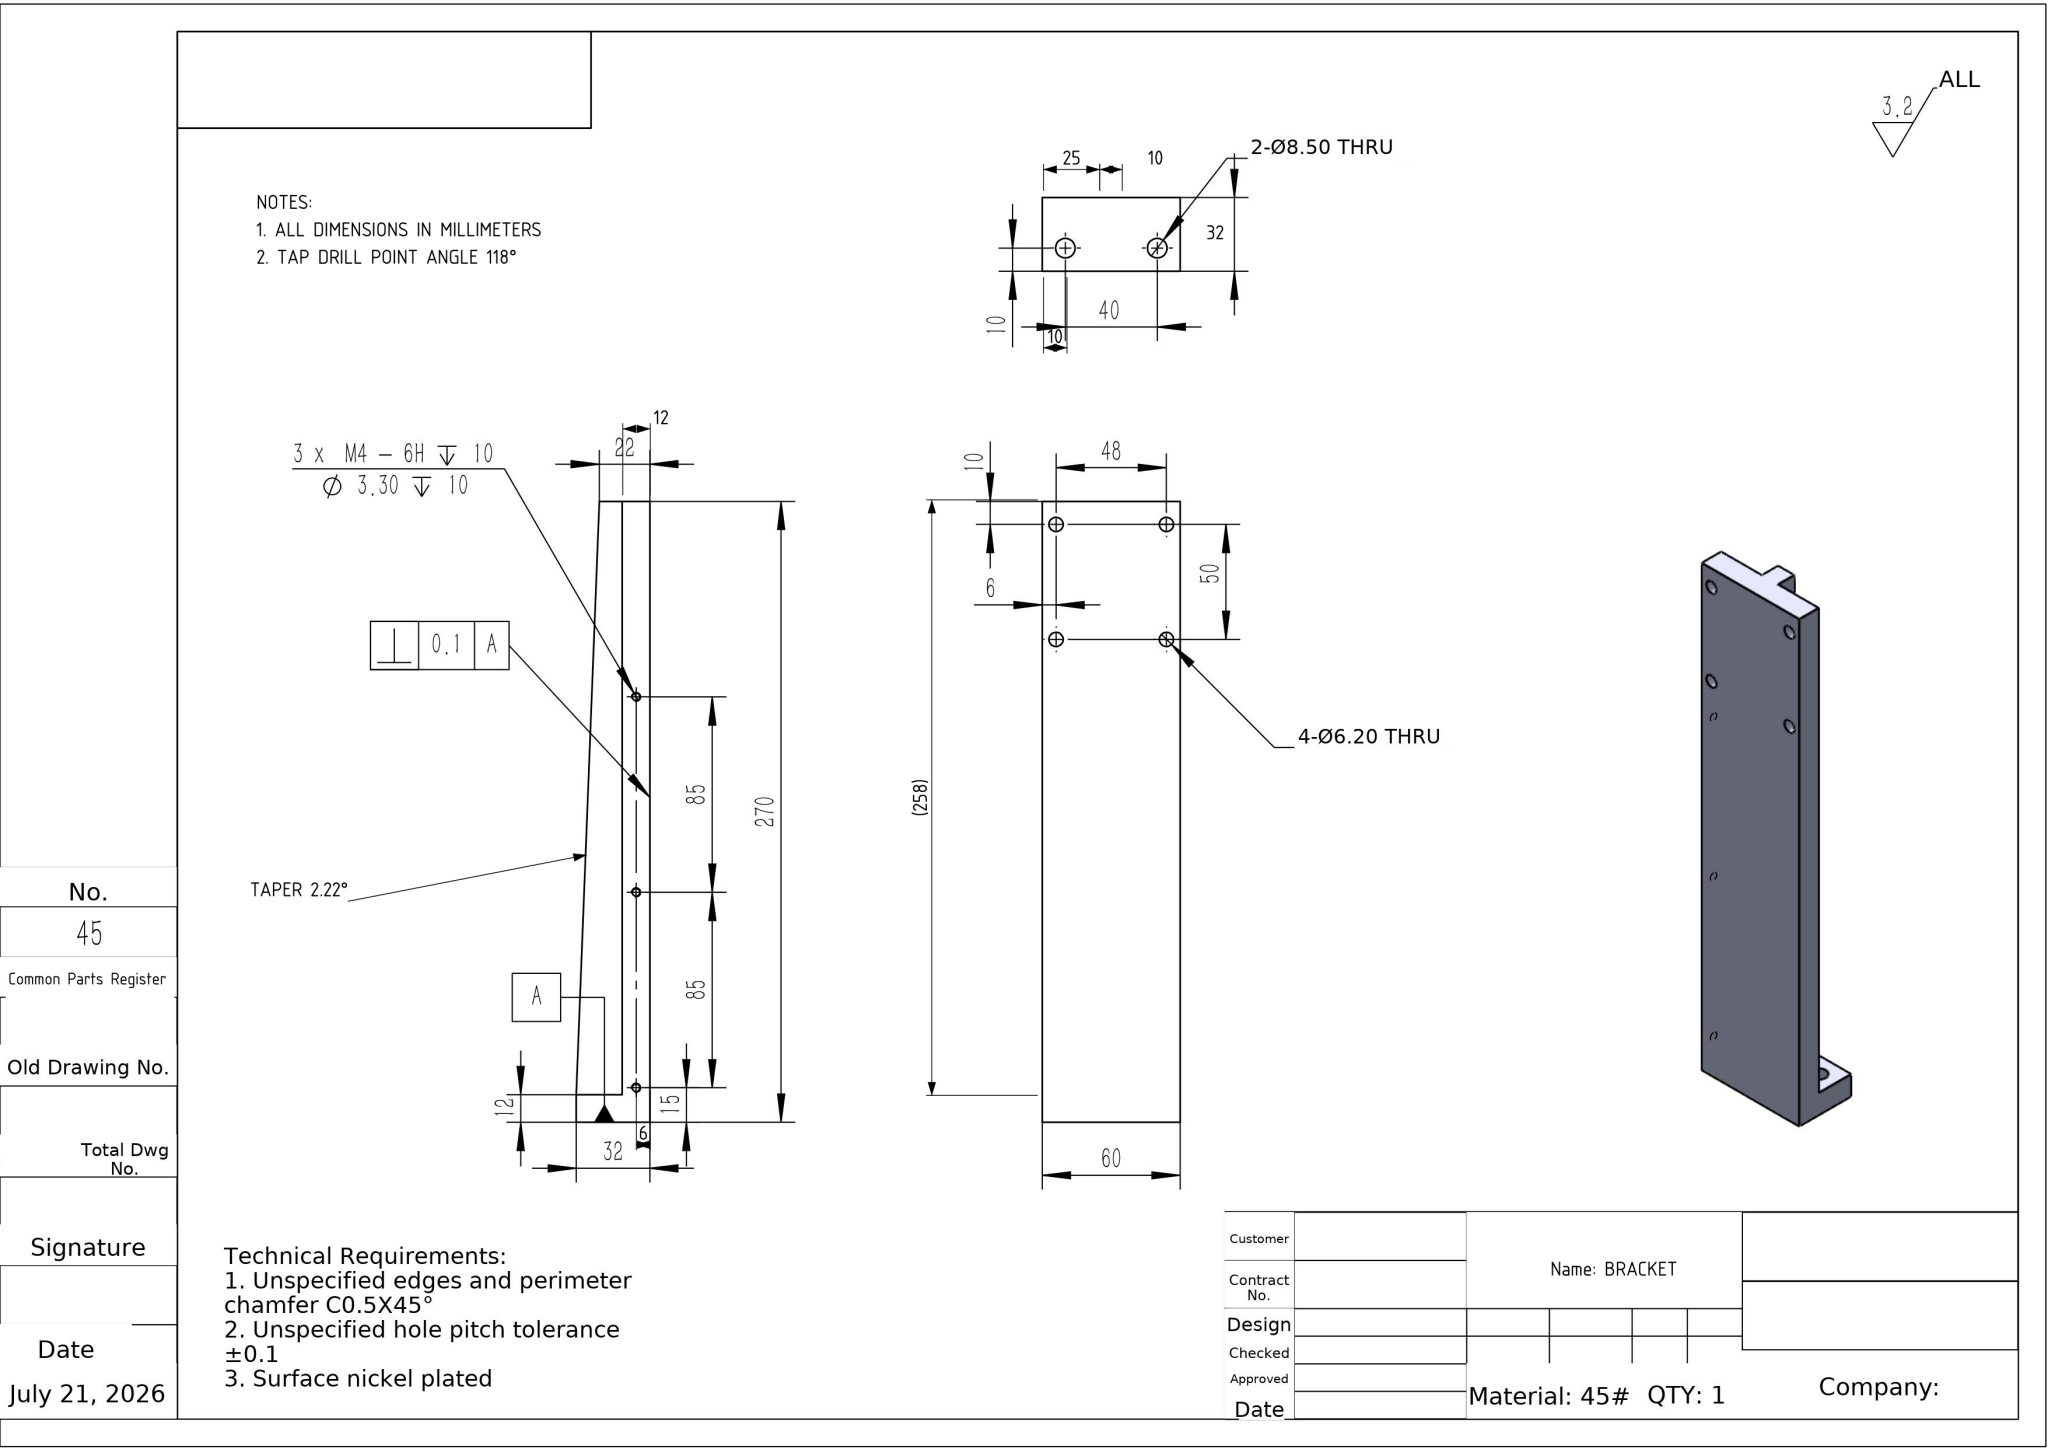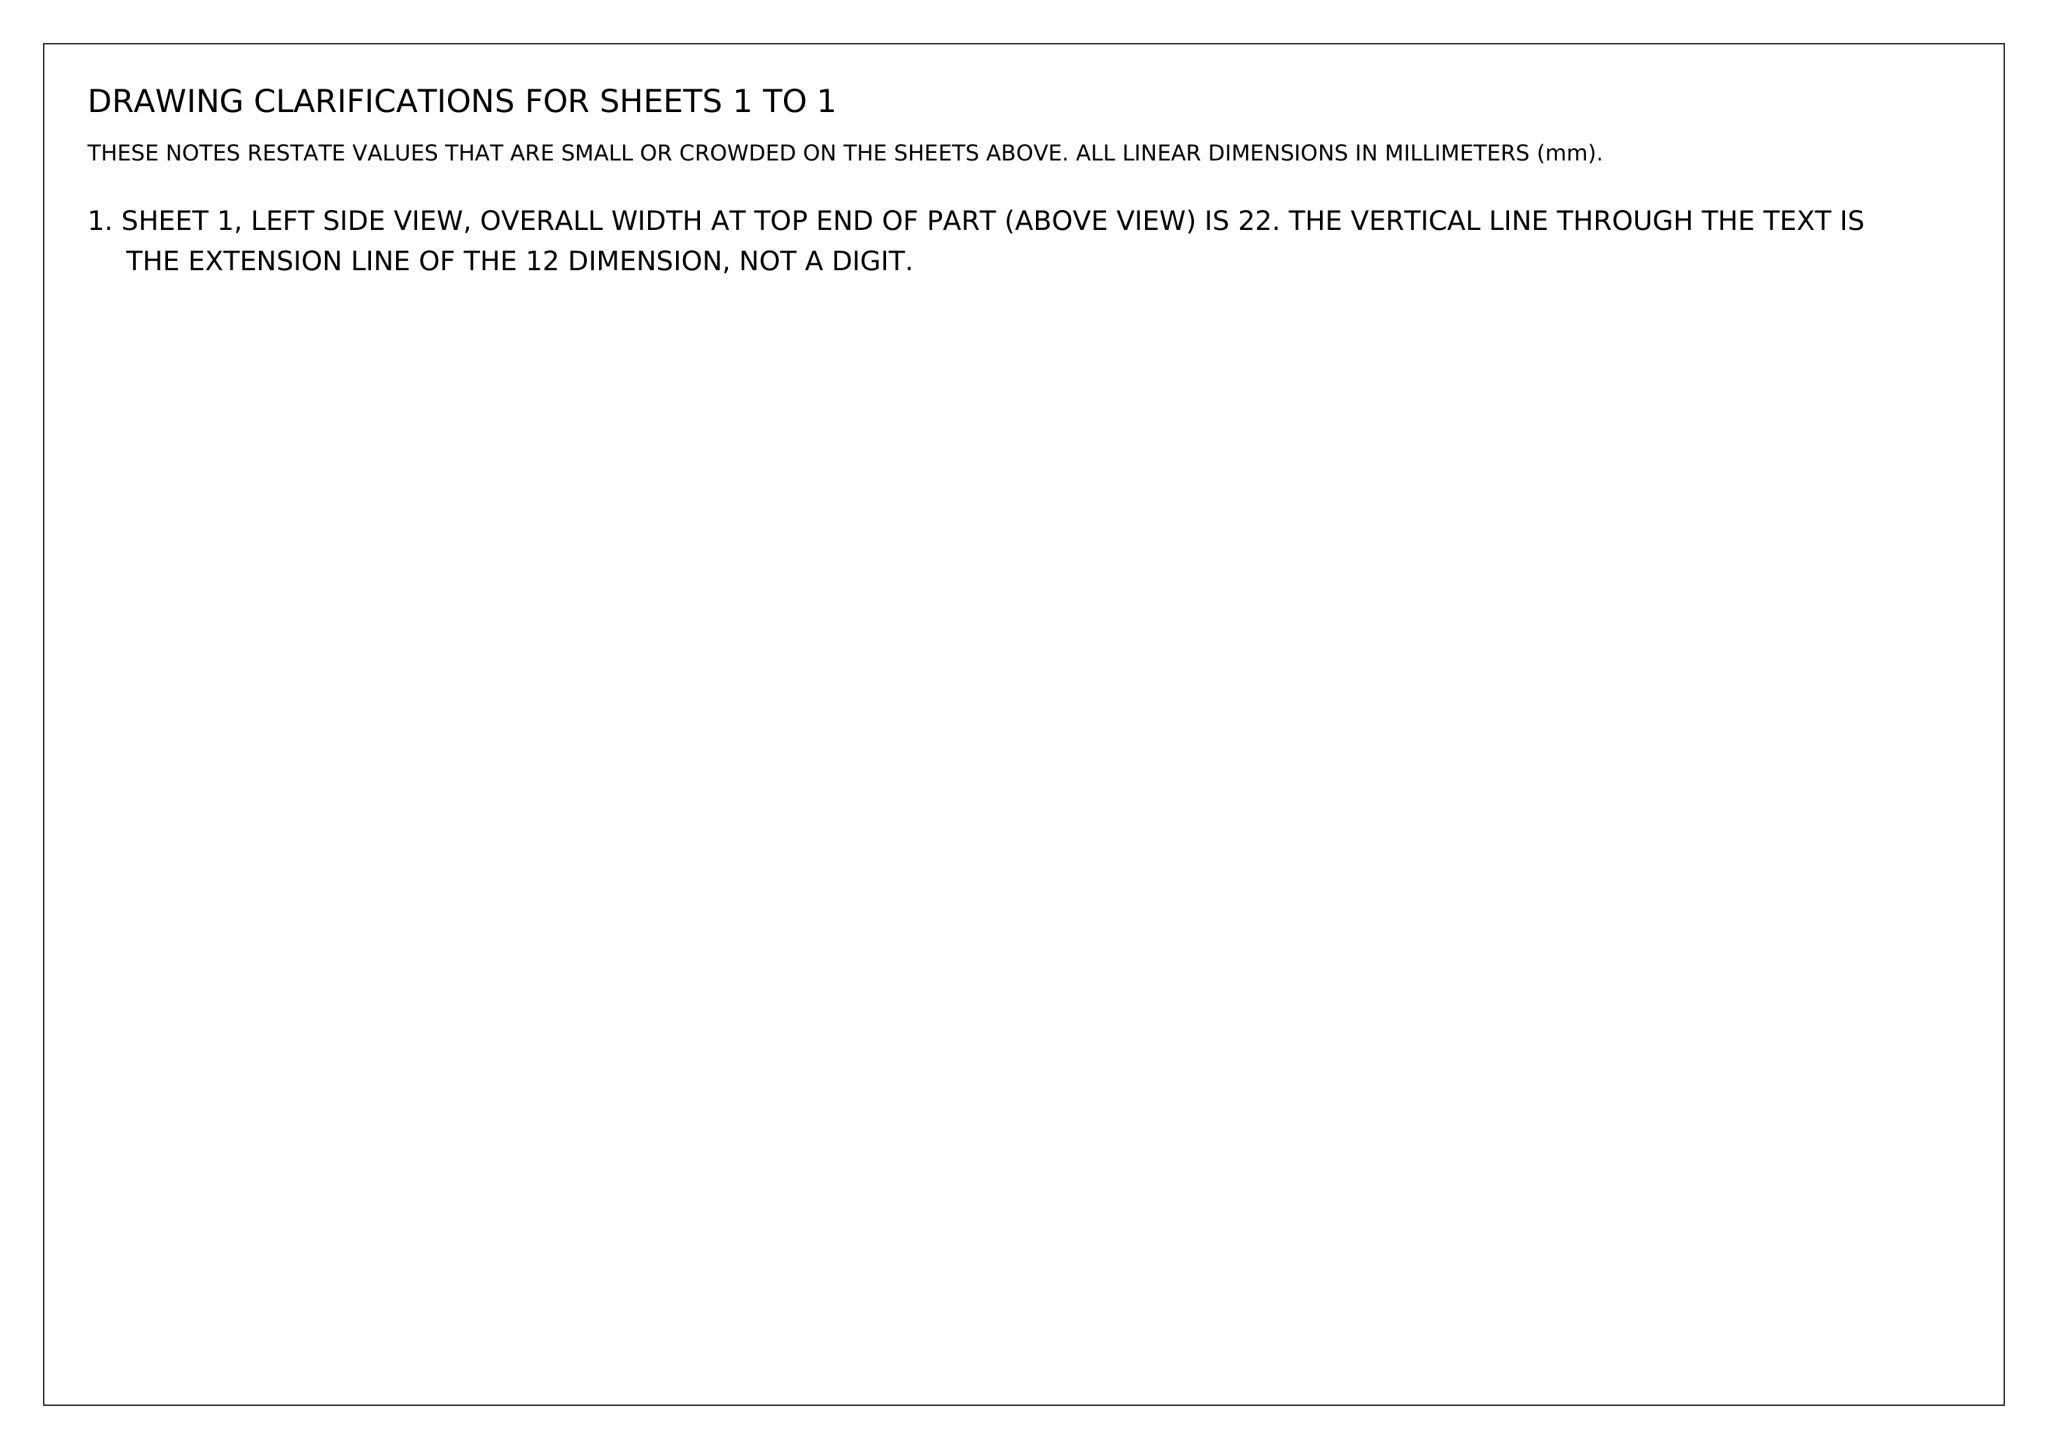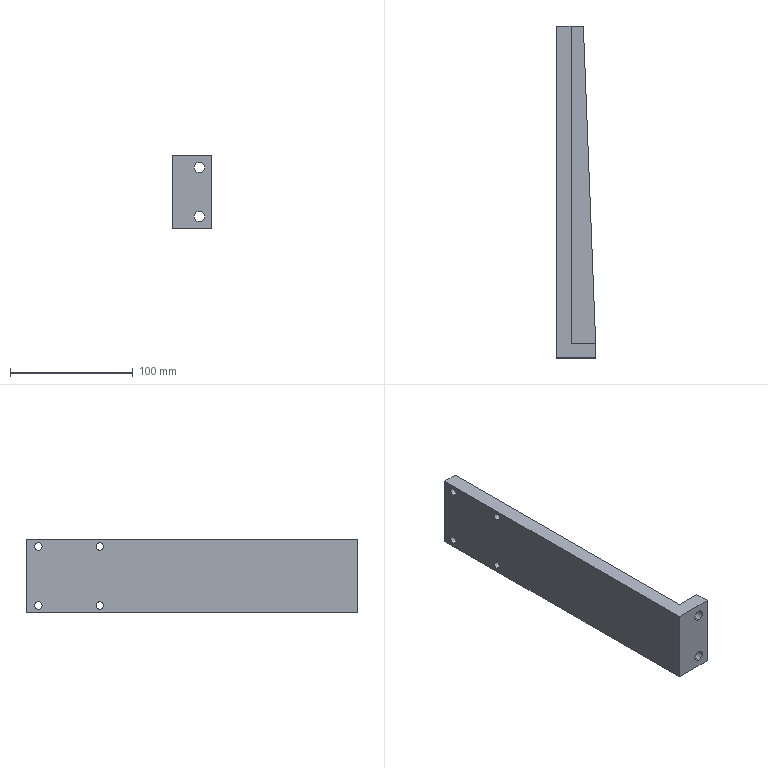Part | NX | mm | 1 solid | 37 faces | box 32 x 270 x 60 mm | volume 244424 mm3 | cylinder 18 | plane 13 | cone 6 | commonest cylinder face diameters 6.2 x8 3.3 x6 8.5 x4